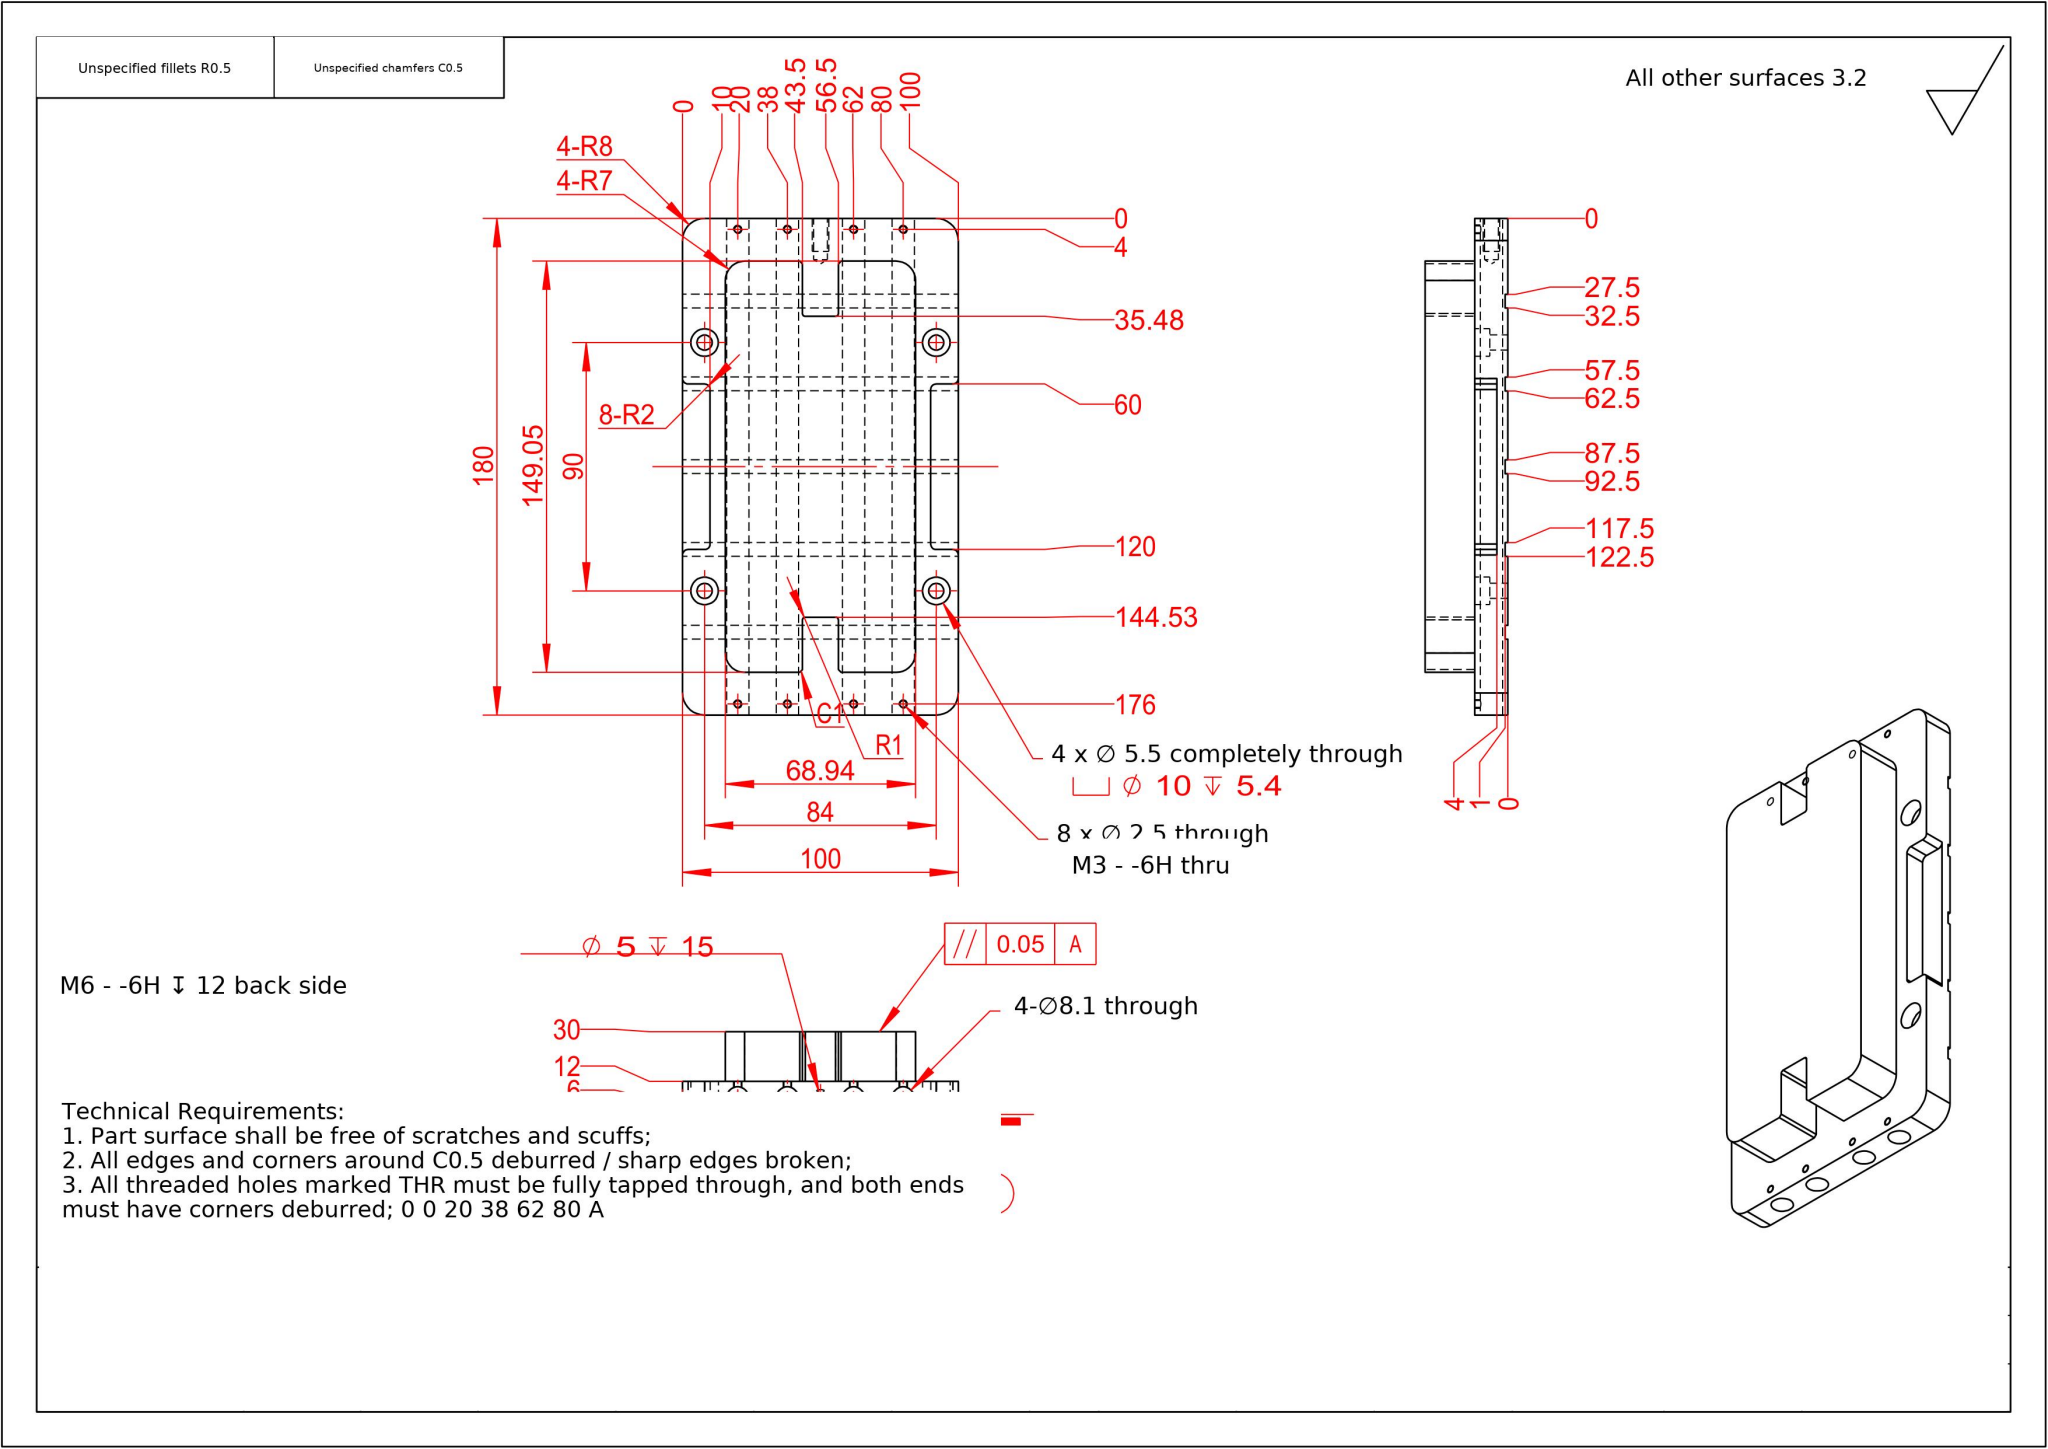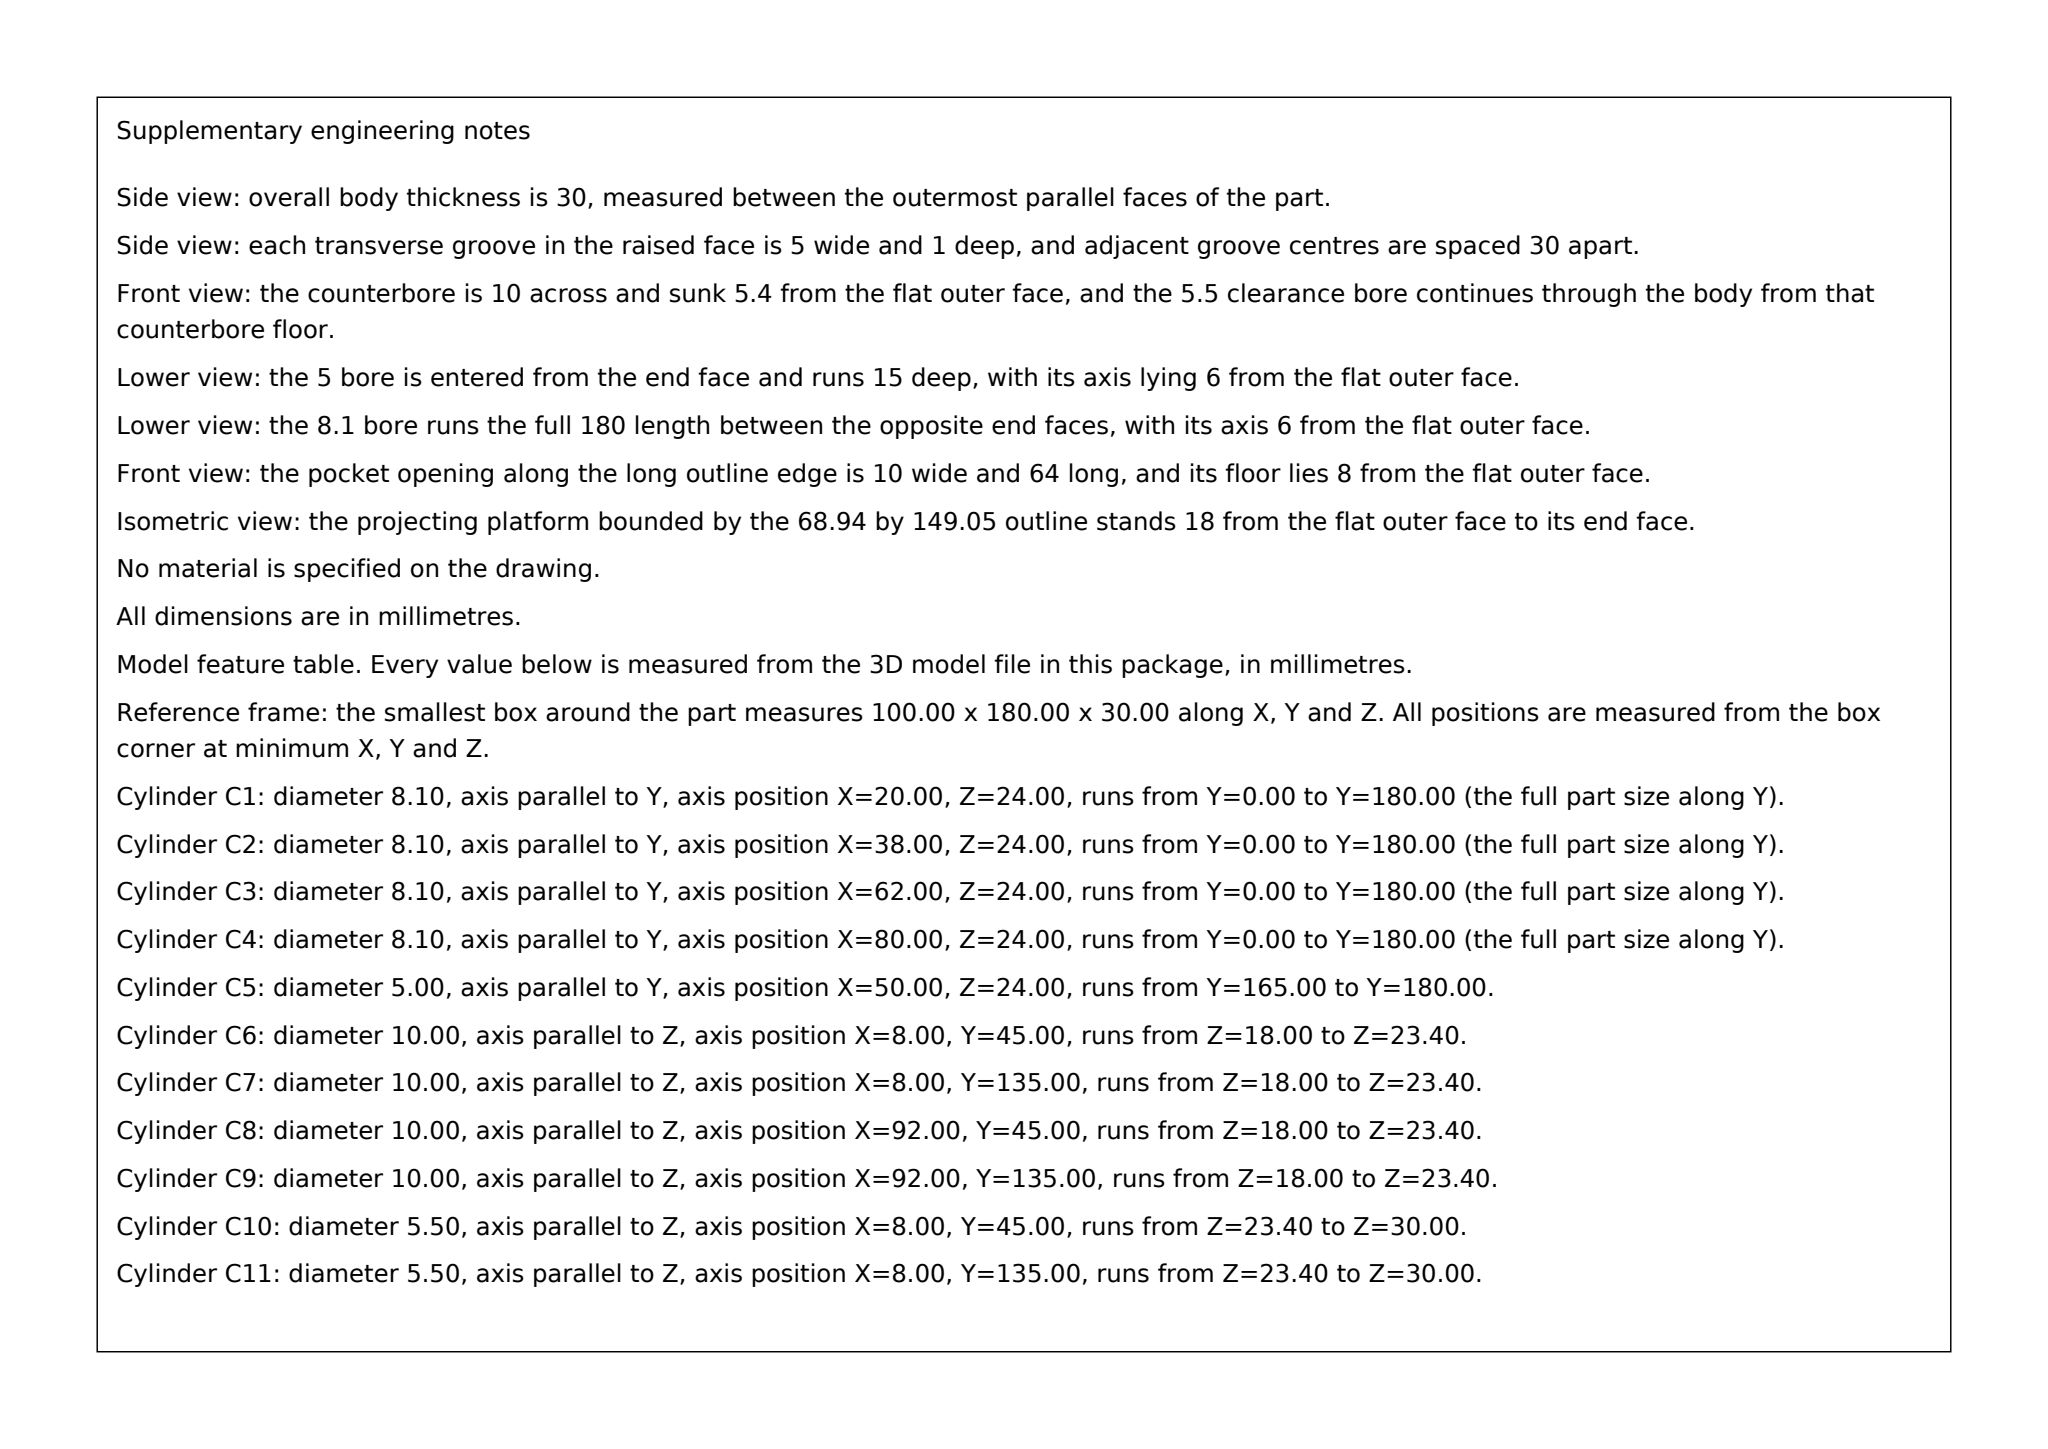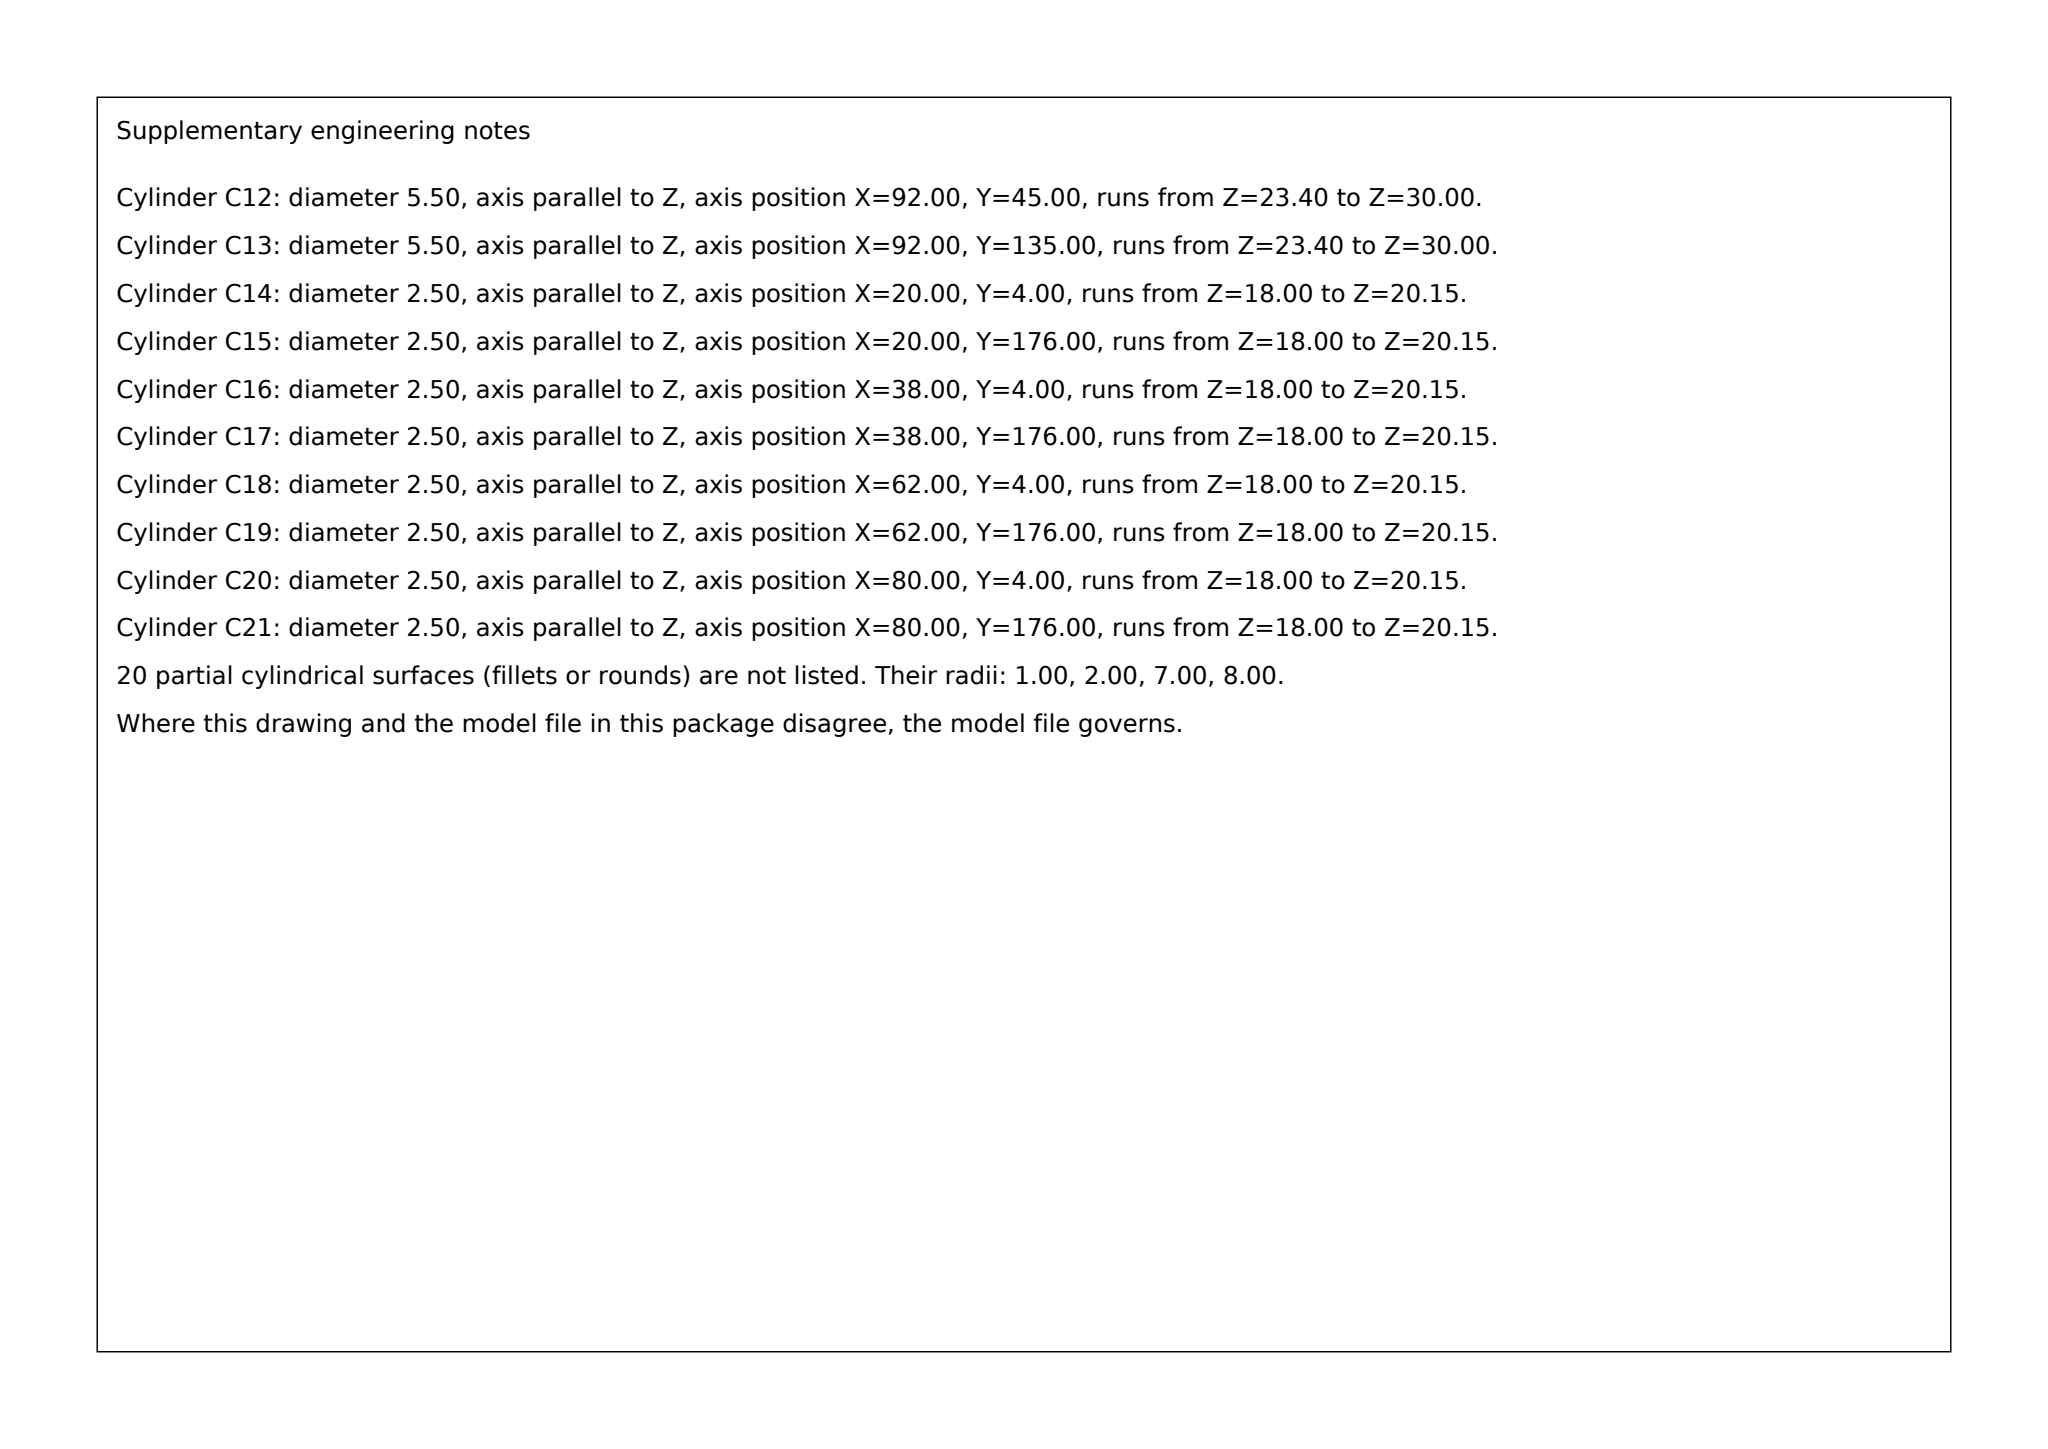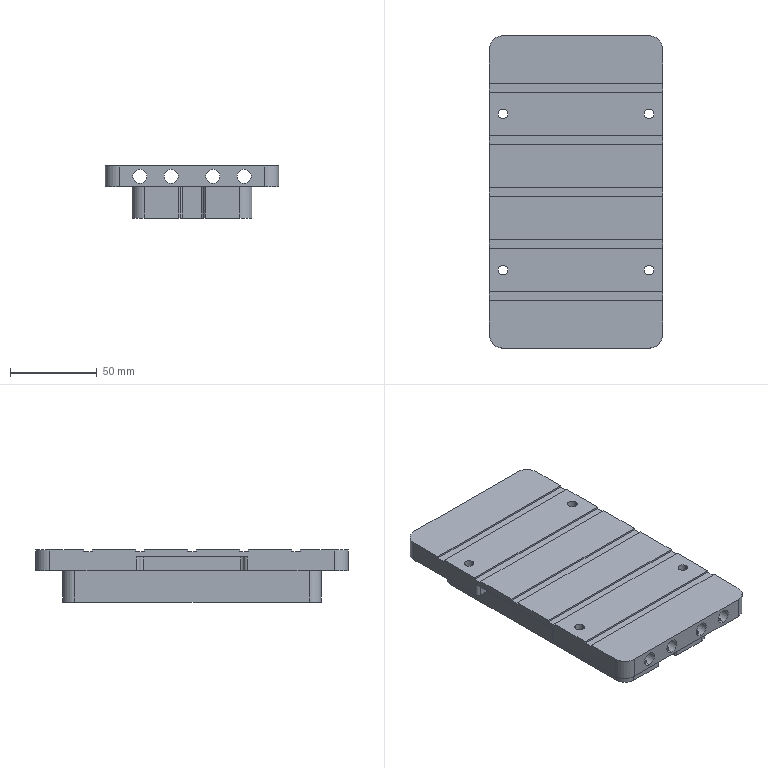Part | SolidWorks | mm | 1 solid | 119 faces | box 100 x 180 x 30 mm | volume 338254 mm3 | cylinder 62 | plane 55 | cone 2 | commonest cylinder face diameters 2.5 x16 10 x8 5.5 x8 8.1 x8 4 x8 16 x4 14 x4 2 x4
Drawing notes:
2X Ø5 DP 15, M6-6H DP 12: BOTH 100X30 END FACES, ON CL, 6 BELOW TOP | from the solid: cyl Ø5 axis y, pos x=50 z=24, len 15, qty 2; bbox 100x180x30, so one in each y=0/y=180 end face, 6 from z=30 face
DATUM A = BACK FACE Z0, OPPOSITE 30 DIM FACE | from the solid: planar faces normal z at offset 0.0 and 30.0; parallelism controls front face rel. to back face
8X Ø2.5 / M3 IN END FLANGE: 2.15 WALL THK ALONG HOLE AXIS | from the solid: Ø2.5 cylinders axis z, length 2.15 at y=4 and y=176, x=20/38/62/80
4 x Ø8.1 THRU: AXIS 6 FROM FRONT FACE (Z0) | from the solid: cyl dia 8.1, axis y, pos (x,z)=(20/38/62/80, 24), len 180; drawing Z0 = STEP z30 face (slot floors z29=Z1, faces z26=Z4), so 30-24=6
5 x GROOVE 5 WIDE x 1 DP IN FRONT FACE, ACROSS FULL 100 | from the solid: y planes 27.5/32.5, 57.5/62.5, 87.5/92.5, 117.5/122.5, 147.5/152.5 (1 face each, full width); 5 floor planes z=29 (1 below z30 face); z=30 split into 6 strips; no x end planes
END FLANGE FACE // FRONT FACE, 2.15 THK; 8 x M3 AT Y4 & Y176 | from the solid: cyl dia 2.5, axis z, len 2.15 at (20/38/62/80, 4) and (20/38/62/80, 176) - axis normal to Z0 face, wall 2.15
4X SIDE EAR (X0-10 AND X90-100, Y60-120): 6.6 THK, OUTER FACE AT Z30, UNDERSIDE AT Z23.4 FROM DATUM A (BACK FACE Z0) | from the solid: axis_planes z=23.4 (count 4) and z=30 with cylinders dia 5.5, axis z, length 6.6 at (8,45),(8,135),(92,45),(92,135)
END FLANGES AT Y4 AND Y176 (8X Ø2.5 / M3): 2.15 THK, FLANGE FACE AT Z26.0 FROM DATUM A (BACK FACE Z0), MATERIAL TO Z28.15 | from the solid: axis_planes z=26.0 (count 2); cylinders dia 2.5, axis z, length 2.15 at x=20,38,62,80 on y=4 and y=176
4X Ø5.5 THRU 6.6 THK EAR; CBORE Ø10 DEPTH 5.4 MEASURED FROM EAR OUTER FACE AT Z30 (OPPOSITE DATUM A), CBORE FLOOR AT Z24.6 | from the solid: cylinders dia 10, axis z, length 5.4 coaxial with dia 5.5 length 6.6 at (8,45),(8,135),(92,45),(92,135); ear faces z=23.4 / z=30
4X SIDE EAR (X0-10 & X90-100, Y60-120) 6.6 THK: OUTER FACE AT Z30, UNDERSIDE AT Z23.4 FROM DATUM A (BACK FACE Z0) | from the solid: Ø5.5 z-cylinders at (8,45),(8,135),(92,45),(92,135) length 6.6; z planes at 23.4 (x4) and 30.0; bbox z = 30
END FLANGES AT Y4 AND Y176 (8X Ø2.5 / M3) 2.15 THK: FLANGE FACE AT Z26.0 FROM DATUM A (BACK FACE Z0), MATERIAL TO Z28.15 | from the solid: Ø2.5 z-cylinders at y4 and y176 length 2.15; z plane at 26.0 (x2)
CBORE Ø10 DP 5.4 MEASURED FROM EAR OUTER FACE AT Z30 (OPPOSITE DATUM A); CBORE FLOOR AT Z24.6 | from the solid: Ø10 z-cylinders length 5.4 coaxial with Ø5.5 holes at (8,45),(8,135),(92,45),(92,135); z plane at 30.0
build123d program:
from build123d import *

# Parameters (mm, degrees)
SKETCH1_W                                       = 100
SKETCH1_H                                       = 180
BOSS_EXTRUDE1_DEPTH                             = 12
FILLET1_R                                       = 8
SKETCH8_R                                       = 4.05
CUT_EXTRUDE2_DEPTH                              = 140
M6_TAPPED_HOLE1_D                               = 5
M6_TAPPED_HOLE1_DEPTH                           = 15
M6_TAPPED_HOLE1_TIP                             = 1.502
SKETCH12_R                                      = 4.05
CUT_EXTRUDE3_DEPTH                              = 140
SKETCH13_R                                      = 4.05
CUT_EXTRUDE4_DEPTH                              = 140
SKETCH15_W                                      = 100
SKETCH15_H                                      = 5
CUT_EXTRUDE6_DEPTH                              = 1
M5_HEX_SOCKET_HEAD_CAP_SCREW_CBORE1_D           = 5.5
M5_HEX_SOCKET_HEAD_CAP_SCREW_CBORE1_CBORE_D     = 10
M5_HEX_SOCKET_HEAD_CAP_SCREW_CBORE1_CBORE_DEPTH = 5.4
M5_HEX_SOCKET_HEAD_CAP_SCREW_CBORE2_D           = 5.5
M5_HEX_SOCKET_HEAD_CAP_SCREW_CBORE2_CBORE_D     = 10
M5_HEX_SOCKET_HEAD_CAP_SCREW_CBORE2_CBORE_DEPTH = 5.4
SKETCH26_R                                      = 4.05
CUT_EXTRUDE7_DEPTH                              = 94
SKETCH28_W                                      = 68.94
SKETCH28_H                                      = 149.05
BOSS_EXTRUDE2_DEPTH                             = 13
FILLET2_R                                       = 7
SKETCH29_W                                      = 10
SKETCH29_H                                      = 60
CUT_EXTRUDE8_DEPTH                              = 8
FILLET3_R                                       = 2
CUT_EXTRUDE9_DEPTH                              = 13
FILLET4_R                                       = 2
SKETCH31_W                                      = 32
SKETCH31_H                                      = 149.05
BOSS_EXTRUDE3_DEPTH                             = 13
BOSS_EXTRUDE4_START                             = 5
BOSS_EXTRUDE4_DEPTH                             = 5
M3_TAPPED_HOLE1_REACH                           = 181.021
M3_TAPPED_HOLE1_BORE_R                          = 1.25
SKETCH37_W                                      = 13
SKETCH37_H                                      = 20
CUT_EXTRUDE10_DEPTH                             = 18
FILLET5_R                                       = 1
CHAMFER1_SIZE                                   = 1


with BuildPart() as part:
    # Sketch1 → Boss-Extrude1 (new body)
    with BuildSketch(Plane.XY):
        with Locations((-28.347, -69.957)):
            Rectangle(SKETCH1_W, SKETCH1_H)
    extrude(amount=BOSS_EXTRUDE1_DEPTH)

    # Fillet1
    fillet1_edges = [part.edges().sort_by_distance(p)[0] for p in [
        (21.653, -159.957, 6),
        (-78.347, -159.957, 6),
        (-78.347, 20.043, 6),
        (21.653, 20.043, 6),
    ]]
    fillet(fillet1_edges, radius=FILLET1_R)

    # Sketch8 → Cut-Extrude2 (cut)
    with BuildSketch(Plane(origin=(0, 20.043, 0), x_dir=(1, 0, 0), z_dir=(0, 1, 0))):
        with Locations(Location((-40.347, -6, 0), (0, 0, 270))):
            Circle(SKETCH8_R)
        with Locations(Location((-16.347, -6, 0), (0, 0, 90))):
            Circle(SKETCH8_R)
    extrude(amount=-CUT_EXTRUDE2_DEPTH, mode=Mode.SUBTRACT)

    # M6 Tapped Hole1
    with Locations(Plane(origin=(0, 20.043, 0), x_dir=(1, 0, 0), z_dir=(0, 1, 0))):
        with Locations((-28.347, -6)):
            Hole(M6_TAPPED_HOLE1_D / 2, depth=M6_TAPPED_HOLE1_DEPTH)
            with Locations((0, 0, -(M6_TAPPED_HOLE1_DEPTH + M6_TAPPED_HOLE1_TIP / 2))):  # 118° drill point
                Cone(0, M6_TAPPED_HOLE1_D / 2, M6_TAPPED_HOLE1_TIP, mode=Mode.SUBTRACT)

    # Sketch12 → Cut-Extrude3 (cut)
    with BuildSketch(Plane(origin=(0, 20.043, 0), x_dir=(1, 0, 0), z_dir=(0, 1, 0))):
        with Locations(Location((-58.347, -6, 0), (0, 0, 270))):
            Circle(SKETCH12_R)
    extrude(amount=-CUT_EXTRUDE3_DEPTH, mode=Mode.SUBTRACT)

    # Sketch13 → Cut-Extrude4 (cut)
    with BuildSketch(Plane(origin=(0, 20.043, 0), x_dir=(1, 0, 0), z_dir=(0, 1, 0))):
        with Locations(Location((1.653, -6, 0), (0, 0, 270))):
            Circle(SKETCH13_R)
    extrude(amount=-CUT_EXTRUDE4_DEPTH, mode=Mode.SUBTRACT)

    # Sketch15 → Cut-Extrude6 (cut)
    with BuildSketch(Plane.XY.offset(12)):
        with Locations((-28.347, -9.957)):
            Rectangle(SKETCH15_W, SKETCH15_H)
        with Locations((-28.347, -39.957)):
            Rectangle(SKETCH15_W, SKETCH15_H)
        with Locations((-28.347, -69.957)):
            Rectangle(SKETCH15_W, SKETCH15_H)
        with Locations((-28.347, -99.957)):
            Rectangle(SKETCH15_W, SKETCH15_H)
        with Locations((-28.347, -129.957)):
            Rectangle(SKETCH15_W, SKETCH15_H)
    extrude(amount=-CUT_EXTRUDE6_DEPTH, mode=Mode.SUBTRACT)

    # M5 Hex Socket Head Cap Screw CBORE1 (through all)
    with Locations(Plane(origin=(0, 0, 0), x_dir=(-1, 0, 0), z_dir=(0, 0, -1))):
        with Locations((70.347, -24.957), (70.347, -114.957)):
            CounterBoreHole(M5_HEX_SOCKET_HEAD_CAP_SCREW_CBORE1_D / 2, M5_HEX_SOCKET_HEAD_CAP_SCREW_CBORE1_CBORE_D / 2, M5_HEX_SOCKET_HEAD_CAP_SCREW_CBORE1_CBORE_DEPTH)

    # M5 Hex Socket Head Cap Screw CBORE2 (through all)
    with Locations(Plane(origin=(0, 0, 0), x_dir=(-1, 0, 0), z_dir=(0, 0, -1))):
        with Locations((-13.653, -24.957), (-13.653, -114.957)):
            CounterBoreHole(M5_HEX_SOCKET_HEAD_CAP_SCREW_CBORE2_D / 2, M5_HEX_SOCKET_HEAD_CAP_SCREW_CBORE2_CBORE_D / 2, M5_HEX_SOCKET_HEAD_CAP_SCREW_CBORE2_CBORE_DEPTH)

    # Sketch26 → Cut-Extrude7 (cut)
    with BuildSketch(Plane(origin=(0, -119.957, 0), x_dir=(1, 0, 0), z_dir=(0, 1, 0))):
        with Locations(Location((-58.347, -6, 0), (0, 0, 270))):
            Circle(SKETCH26_R)
        with Locations(Location((-40.347, -6, 0), (0, 0, 270))):
            Circle(SKETCH26_R)
        with Locations(Location((-16.347, -6, 0), (0, 0, 270))):
            Circle(SKETCH26_R)
        with Locations(Location((1.653, -6, 0), (0, 0, 270))):
            Circle(SKETCH26_R)
    extrude(amount=-CUT_EXTRUDE7_DEPTH, mode=Mode.SUBTRACT)

    # Sketch28 → Boss-Extrude2 (add)
    with BuildSketch(Plane(origin=(0, 0, 0), x_dir=(-1, 0, 0), z_dir=(0, 0, -1))):
        with Locations((28.347, -69.957)):
            Rectangle(SKETCH28_W, SKETCH28_H)
    extrude(amount=BOSS_EXTRUDE2_DEPTH)

    # Fillet2
    fillet2_edges = [part.edges().sort_by_distance(p)[0] for p in [
        (-62.817, -144.482, -6.5),
        (-62.817, 4.568, -6.5),
        (6.123, 4.568, -6.5),
        (6.123, -144.482, -6.5),
    ]]
    fillet(fillet2_edges, radius=FILLET2_R)

    # Sketch29 → Cut-Extrude8 (cut)
    with BuildSketch(Plane(origin=(0, 0, 0), x_dir=(-1, 0, 0), z_dir=(0, 0, -1))):
        with Locations((73.347, -69.957)):
            Rectangle(SKETCH29_W, SKETCH29_H)
        with Locations((-16.653, -69.957)):
            Rectangle(SKETCH29_W, SKETCH29_H)
    extrude(amount=-CUT_EXTRUDE8_DEPTH, mode=Mode.SUBTRACT)

    # Fillet3
    fillet3_edges = [part.edges().sort_by_distance(p)[0] for p in [
        (-78.347, -39.957, 4),
        (-78.347, -99.957, 4),
        (-68.347, -99.957, 4),
        (-68.347, -39.957, 4),
        (21.653, -39.957, 4),
        (11.653, -39.957, 4),
        (11.653, -99.957, 4),
        (21.653, -99.957, 4),
    ]]
    fillet(fillet3_edges, radius=FILLET3_R)

    # Sketch30 → Cut-Extrude9 (cut)
    with BuildSketch(Plane(origin=(0, 0, -13), x_dir=(-1, 0, 0), z_dir=(0, 0, -1))):
        Polygon((12.347, 4.568), (44.347, 4.568), (28.347, -4.669), align=None)
        Polygon((28.347, -135.244), (12.347, -144.482), (44.347, -144.482), align=None)
    extrude(amount=-CUT_EXTRUDE9_DEPTH, mode=Mode.SUBTRACT)

    # Fillet4
    fillet4_edges = [part.edges().sort_by_distance(p)[0] for p in [
        (-28.347, -4.669, -6.5),
    ]]
    fillet(fillet4_edges, radius=FILLET4_R)

    # Sketch31 → Boss-Extrude3 (add)
    with BuildSketch(Plane(origin=(0, 0, -13), x_dir=(-1, 0, 0), z_dir=(0, 0, -1))):
        with Locations((28.347, -69.957)):
            Rectangle(SKETCH31_W, SKETCH31_H)
    extrude(amount=-BOSS_EXTRUDE3_DEPTH)

    # Sketch34 → Boss-Extrude4 (add)
    with BuildSketch(Plane(origin=(0, 0, -13), x_dir=(-1, 0, 0), z_dir=(0, 0, -1)).offset(BOSS_EXTRUDE4_START)):
        with BuildLine():
            Line((55.817, 4.568), (0.8771, 4.568))
            ThreePointArc((0.8771, 4.568), (-4.073, 2.518), (-6.123, -2.432))
            Line((-6.123, -2.432), (-6.123, -137.482))
            ThreePointArc((-6.123, -137.482), (-4.073, -142.431), (0.8771, -144.482))
            Line((0.8771, -144.482), (55.817, -144.482))
            ThreePointArc((55.817, -144.482), (60.767, -142.431), (62.817, -137.482))
            Line((62.817, -137.482), (62.817, -2.432))
            ThreePointArc((62.817, -2.432), (60.767, 2.518), (55.817, 4.568))
        make_face()
    extrude(amount=-BOSS_EXTRUDE4_DEPTH)

    # M3 Tapped Hole1 bore → M3 Tapped Hole1 (cut, up to next)
    with BuildSketch(Plane(origin=(0, 0, 0), x_dir=(-1, 0, 0), z_dir=(0, 0, -1)), mode=Mode.PRIVATE) as m3_tapped_hole1_sk1:
        with Locations((58.347, 16.043)):
            Circle(M3_TAPPED_HOLE1_BORE_R)
    m3_tapped_hole1_tool1 = extrude(m3_tapped_hole1_sk1.sketch, amount=-M3_TAPPED_HOLE1_REACH, mode=Mode.PRIVATE) & part.part
    # M3 Tapped Hole1 bore → M3 Tapped Hole1 (cut, up to next)
    with BuildSketch(Plane(origin=(0, 0, 0), x_dir=(-1, 0, 0), z_dir=(0, 0, -1)), mode=Mode.PRIVATE) as m3_tapped_hole1_sk2:
        with Locations((40.347, 16.043)):
            Circle(M3_TAPPED_HOLE1_BORE_R)
    m3_tapped_hole1_tool2 = extrude(m3_tapped_hole1_sk2.sketch, amount=-M3_TAPPED_HOLE1_REACH, mode=Mode.PRIVATE) & part.part
    # M3 Tapped Hole1 bore → M3 Tapped Hole1 (cut, up to next)
    with BuildSketch(Plane(origin=(0, 0, 0), x_dir=(-1, 0, 0), z_dir=(0, 0, -1)), mode=Mode.PRIVATE) as m3_tapped_hole1_sk3:
        with Locations((16.347, 16.043)):
            Circle(M3_TAPPED_HOLE1_BORE_R)
    m3_tapped_hole1_tool3 = extrude(m3_tapped_hole1_sk3.sketch, amount=-M3_TAPPED_HOLE1_REACH, mode=Mode.PRIVATE) & part.part
    # M3 Tapped Hole1 bore → M3 Tapped Hole1 (cut, up to next)
    with BuildSketch(Plane(origin=(0, 0, 0), x_dir=(-1, 0, 0), z_dir=(0, 0, -1)), mode=Mode.PRIVATE) as m3_tapped_hole1_sk4:
        with Locations((-1.653, 16.043)):
            Circle(M3_TAPPED_HOLE1_BORE_R)
    m3_tapped_hole1_tool4 = extrude(m3_tapped_hole1_sk4.sketch, amount=-M3_TAPPED_HOLE1_REACH, mode=Mode.PRIVATE) & part.part
    m3_tapped_hole1_1 = m3_tapped_hole1_tool1.solids().sort_by_distance((-58.347, 16.043, 0))[0]
    add(m3_tapped_hole1_1, mode=Mode.SUBTRACT)
    m3_tapped_hole1_2 = m3_tapped_hole1_tool2.solids().sort_by_distance((-40.347, 16.043, 0))[0]
    add(m3_tapped_hole1_2, mode=Mode.SUBTRACT)
    m3_tapped_hole1_3 = m3_tapped_hole1_tool3.solids().sort_by_distance((-16.347, 16.043, 0))[0]
    add(m3_tapped_hole1_3, mode=Mode.SUBTRACT)
    m3_tapped_hole1_4 = m3_tapped_hole1_tool4.solids().sort_by_distance((1.653, 16.043, 0))[0]
    add(m3_tapped_hole1_4, mode=Mode.SUBTRACT)
    m3_tapped_hole1 = m3_tapped_hole1_1 + m3_tapped_hole1_2 + m3_tapped_hole1_3 + m3_tapped_hole1_4  # M3 Tapped Hole1 as one shape, for the pattern or mirror that repeats it

    # Mirror1: M3 Tapped Hole1 across plane
    add(m3_tapped_hole1.mirror(Plane.ZX.offset(-69.957)), mode=Mode.SUBTRACT)

    # Sketch37 → Cut-Extrude10 (cut)
    with BuildSketch(Plane(origin=(0, 0, -18), x_dir=(-1, 0, 0), z_dir=(0, 0, -1))):
        with Locations((28.347, -5.432)):
            Rectangle(SKETCH37_W, SKETCH37_H)
        with Locations((28.347, -134.482)):
            Rectangle(SKETCH37_W, SKETCH37_H)
    extrude(amount=-CUT_EXTRUDE10_DEPTH, mode=Mode.SUBTRACT)

    # Fillet5
    fillet5_edges = [part.edges().sort_by_distance(p)[0] for p in [
        (-34.847, -15.432, -9),
        (-21.847, -15.432, -9),
        (-34.847, -124.482, -9),
        (-21.847, -124.482, -9),
    ]]
    fillet(fillet5_edges, radius=FILLET5_R)

    # Chamfer1
    chamfer1_edges = [part.edges().sort_by_distance(p)[0] for p in [
        (-34.847, 4.568, -9),
        (-21.847, 4.568, -9),
        (-34.847, -144.482, -9),
        (-21.847, -144.482, -9),
    ]]
    chamfer(chamfer1_edges, length=CHAMFER1_SIZE)


solid = part.part